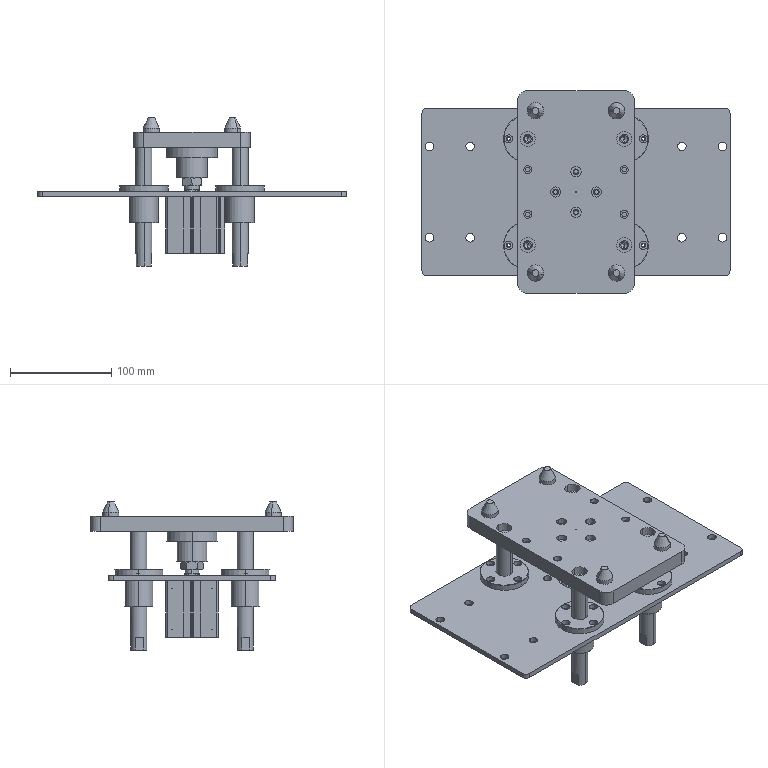Assembly | SolidWorks | mm | 18 component files | 18 solids | 743 faces | box 304 x 200 x 146 mm | volume 890172 mm3 | cylinder 400 | plane 201 | cone 140 | spline 2 | commonest cylinder face diameters 0.4 x46 8 x40 4.5 x40 16 x36 3.3 x32 10 x28 8.5 x24 6.647 x16
Bill of materials:
DC-46-014 | 1 |  | Thin, flat rectangular plate with small corner radii and a symmetric pattern of through holes: one large central hole surrounded by four holes, four medium holes each ringed by four small holes, and eight holes in two rows near the long edges.
DC-46-015 | 4 |  | Long, slender cylindrical tube or sleeve with a concentric bore at one end. A short section at the other end has a slightly smaller diameter, and that end looks angled or chamfered.
DC-46-016 | 4 |  | Solid round part: a short cylindrical base topped by a cone-shaped section (frustum) with a flat circular top.
DC-46-017 | 1 |  | Thick rectangular plate with rounded corners and 16 through holes in a symmetric layout: four counterbored corner holes, four larger plain holes, and eight smaller holes.
DC-46-018 | 1 |  | Flanged bushing-like part: a thick round flange with four through holes evenly spaced on a circle, a central through bore, and a smaller-diameter cylindrical spigot.
LMF16UU(FlangedLinearBearing) | 4 |  | Flanged sleeve: a thin round flange with four holes evenly spaced on a circle, a large central bore, and a long cylindrical spigot. Edges have small chamfers.
SDA-40- M14x1.5-1-dx | 1 |  | Hexagonal nut-like body with a plain central round bore and chamfered corners on both faces.
SDAS-40x2020_b-1-dx | 1 |  | Square, extruded-looking block with four counterbored through holes at the corners, slots running the full length of the side faces, a raised round boss with a central bore on the top face inside a circular groove, and a side boss with two round openings.
SDAS-40x20-B20_r-1-dx | 1 |  | Stepped cylindrical pin: a large disc-shaped head, a middle shaft, a narrow groove or neck with a small local cut, and a smaller-diameter tip with a chamfer.
Mates:
1. concentric | DC-46-014-4 face at (311.865, 195.227, 1950.133) dir (0, 0, 1) r 17.5 | SDA40x20SB_0_+_-1-1/SDAS-40x20-B20_r-1-dx-1 face at (311.865, 195.227, 2027.133) dir (0, 0, 1) r 7
2. coincident | DC-46-014-4 face at (311.865, 195.227, 2027.133) dir (0, 0, -1) | SDA40x20SB_0_+_-1-1/SDAS-40x2020_b-1-dx-1 edge at (303.465, 169.227, 2027.133) dir (-1, 0, 0)
3. parallel | DC-46-014-4 face at (463.865, 112.727, 2032.133) dir (0, -1, 0) | SDA40x20SB_0_+_-1-1/SDAS-40x2020_b-1-dx-1 face at (303.465, 169.227, 1971.133) dir (0, -1, 0)
4. concentric | DC-46-014-4 face at (359.365, 142.727, 2109.133) dir (0, 0, -1) r 14.1 | LMF16UU(FlangedLinearBearing)-1 face at (359.365, 142.727, 2001.133) dir (0, 0, 1) r 14
5. coincident | DC-46-014-4 face at (311.865, 195.227, 2032.133) dir (0, 0, 1) | LMF16UU(FlangedLinearBearing)-1 face at (359.365, 142.727, 2032.133) dir (0, 0, -1)
6. concentric | DC-46-014-4 edge at (359.365, 247.727, 2032.133) dir (0, 0, 1) r 14.1 | LMF16UU(FlangedLinearBearing)-2 face at (359.365, 247.727, 2001.133) dir (0, 0, 1) r 14
7. coincident | LMF16UU(FlangedLinearBearing)-1 face at (359.365, 142.727, 2038.133) dir (0, 0, 1) | LMF16UU(FlangedLinearBearing)-2 face at (359.365, 247.727, 2038.133) dir (0, 0, 1)
8. concentric | DC-46-014-4 face at (264.365, 247.727, 2109.133) dir (0, 0, -1) r 14.1 | LMF16UU(FlangedLinearBearing)-3 face at (264.365, 247.727, 2001.133) dir (0, 0, 1) r 14
9. coincident | LMF16UU(FlangedLinearBearing)-2 face at (359.365, 247.727, 2038.133) dir (0, 0, 1) | LMF16UU(FlangedLinearBearing)-3 face at (264.365, 247.727, 2038.133) dir (0, 0, 1)
10. concentric | DC-46-014-4 face at (264.365, 142.727, 2109.133) dir (0, 0, -1) r 14.1 | LMF16UU(FlangedLinearBearing)-4 face at (264.365, 142.727, 2001.133) dir (0, 0, 1) r 14
11. coincident | LMF16UU(FlangedLinearBearing)-3 face at (264.365, 247.727, 2038.133) dir (0, 0, 1) | LMF16UU(FlangedLinearBearing)-4 face at (264.365, 142.727, 2038.133) dir (0, 0, 1)
12. parallel | DC-46-014-4 face at (463.865, 277.727, 2032.133) dir (0, 1, 0) | LMF16UU(FlangedLinearBearing)-2 plane at (359.365, 247.727, 2019.633) dir (0, 1, 0)
13. parallel | DC-46-014-4 face at (463.865, 112.727, 2032.133) dir (0, -1, 0) | LMF16UU(FlangedLinearBearing)-1 plane at (359.365, 142.727, 2019.633) dir (0, 1, 0)
14. parallel | DC-46-014-4 face at (463.865, 277.727, 2032.133) dir (0, 1, 0) | LMF16UU(FlangedLinearBearing)-3 plane at (264.365, 247.727, 2019.633) dir (0, 1, 0)
15. parallel | DC-46-014-4 face at (463.865, 112.727, 2032.133) dir (0, -1, 0) | LMF16UU(FlangedLinearBearing)-4 plane at (264.365, 142.727, 2019.633) dir (0, 1, 0)
16. concentric | SDA40x20SB_0_+_-1-1/SDAS-40x20-B20_r-1-dx-1 face at (311.865, 195.227, 2027.133) dir (0, 0, 1) r 7 | DC-46-017-1 face at (311.865, 195.227, 2075.633) dir (0, 0, -1) r 0.095
17. concentric | SDA40x20SB_0_+_-1-1/SDAS-40x20-B20_r-1-dx-1 face at (311.865, 195.227, 2027.133) dir (0, 0, 1) r 7 | DC-46-018-1 face at (311.865, 195.227, 2045.633) dir (0, 0, 1) r 15
18. parallel | DC-46-014-4 face at (463.865, 277.727, 2032.133) dir (0, 1, 0) | DC-46-018-1 plane at (311.865, 195.227, 2075.633) dir (0, 1, 0)
19. coincident | DC-46-017-1 face at (311.865, 195.227, 2075.633) dir (0, 0, -1) | DC-46-018-1 face at (311.865, 195.227, 2075.633) dir (0, 0, 1)
20. concentric | LMF16UU(FlangedLinearBearing)-3 face at (264.365, 247.727, 2001.133) dir (0, 0, 1) r 8 | DC-46-015-1 face at (264.365, 247.727, 2078.633) dir (0, 0, -1) r 8
21. coincident | DC-46-017-1 edge at (264.365, 247.727, 2078.633) dir (0, 0, 1) r 4.5 | DC-46-015-1 face at (264.365, 247.727, 2078.633) dir (0, 0, 1)
22. concentric | LMF16UU(FlangedLinearBearing)-4 face at (264.365, 142.727, 2001.133) dir (0, 0, 1) r 8 | DC-46-015-2 face at (264.365, 142.727, 2078.633) dir (0, 0, -1) r 8
23. coincident | DC-46-015-1 face at (264.365, 247.727, 1958.633) dir (0, 0, -1) | DC-46-015-2 face at (264.365, 142.727, 1958.633) dir (0, 0, -1)
24. concentric | LMF16UU(FlangedLinearBearing)-2 face at (359.365, 247.727, 2001.133) dir (0, 0, 1) r 8 | DC-46-015-3 face at (359.365, 247.727, 2078.633) dir (0, 0, -1) r 8
25. coincident | DC-46-015-1 face at (264.365, 247.727, 1958.633) dir (0, 0, -1) | DC-46-015-3 face at (359.365, 247.727, 1958.633) dir (0, 0, -1)
26. concentric | LMF16UU(FlangedLinearBearing)-1 face at (359.365, 142.727, 2001.133) dir (0, 0, 1) r 8 | DC-46-015-4 face at (359.365, 142.727, 2078.633) dir (0, 0, -1) r 8
27. coincident | DC-46-015-2 face at (264.365, 142.727, 1958.633) dir (0, 0, -1) | DC-46-015-4 face at (359.365, 142.727, 1958.633) dir (0, 0, -1)
28. concentric | DC-46-017-1 face at (271.865, 115.227, 2088.633) dir (0, 0, 1) r 8 | DC-46-016-1 face at (271.865, 115.227, 2104.633) dir (0, 0, -1) r 7.95
29. coincident | DC-46-017-1 face at (271.865, 115.227, 2088.633) dir (0, 0, 1) | DC-46-016-1 face at (271.865, 115.227, 2088.633) dir (0, 0, -1)
30. concentric | DC-46-017-1 face at (271.865, 275.227, 2088.633) dir (0, 0, 1) r 8 | DC-46-016-2 face at (271.865, 275.227, 2104.633) dir (0, 0, -1) r 7.95
31. coincident | DC-46-017-1 face at (271.865, 275.227, 2088.633) dir (0, 0, 1) | DC-46-016-2 edge at (271.865, 275.227, 2088.633) dir (0, 0, 1) r 7.95
32. concentric | DC-46-017-1 face at (351.865, 275.227, 2088.633) dir (0, 0, 1) r 8 | DC-46-016-3 face at (351.865, 275.227, 2104.633) dir (0, 0, -1) r 7.95
33. coincident | DC-46-017-1 face at (351.865, 275.227, 2088.633) dir (0, 0, 1) | DC-46-016-3 edge at (351.865, 275.227, 2088.633) dir (0, 0, 1) r 7.95
34. concentric | DC-46-017-1 face at (351.865, 115.227, 2088.633) dir (0, 0, 1) r 8 | DC-46-016-4 face at (351.865, 115.227, 2104.633) dir (0, 0, -1) r 7.95
35. coincident | DC-46-017-1 face at (351.865, 115.227, 2088.633) dir (0, 0, 1) | DC-46-016-4 edge at (351.865, 115.227, 2088.633) dir (0, 0, 1) r 7.95
36. parallel | DC-46-014-4 edge at (463.865, 117.727, 2032.133) dir (0, 1, 0) | DC-46-017-1 face at (369.365, 295.227, 2090.633) dir (1, 0, 0)
37. distance | DC-46-018-1 face at (311.865, 195.227, 2045.633) dir (0, 0, -1) | SDA40x20SB_0_+_-1-1/SDA-40- M14x1.5-1-dx-1 face at (311.865, 195.227, 2037.633) dir (0, 0, -1)